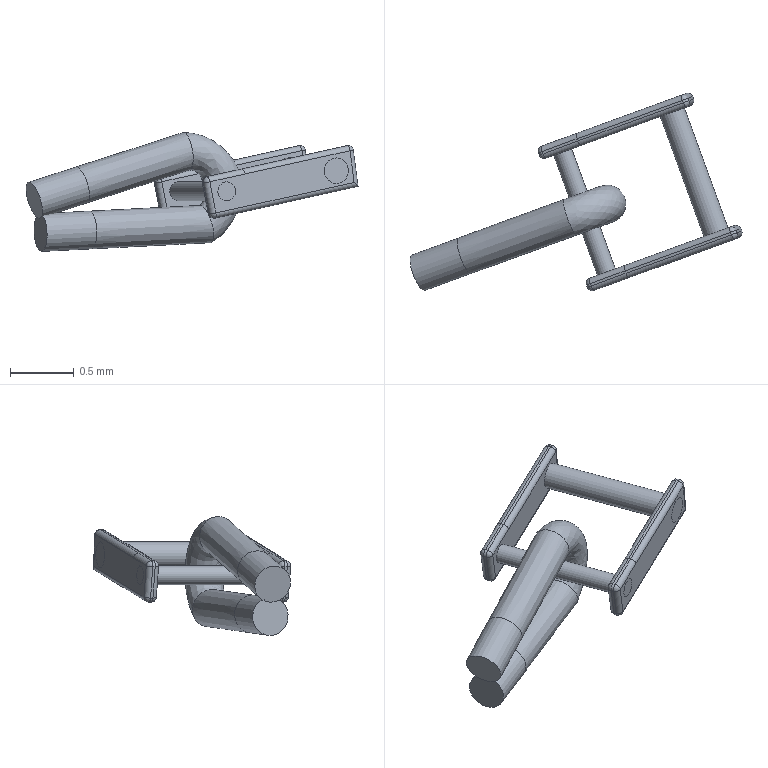Component | NX | MODEL11_2 | 5 solids | 70 faces | volume 0 mm3 | cylinder 35 | plane 20 | sphere 12 | spline 3 | commonest cylinder face diameters 0.08 x26 0.148 x4 0.2 x3 0.296 x2